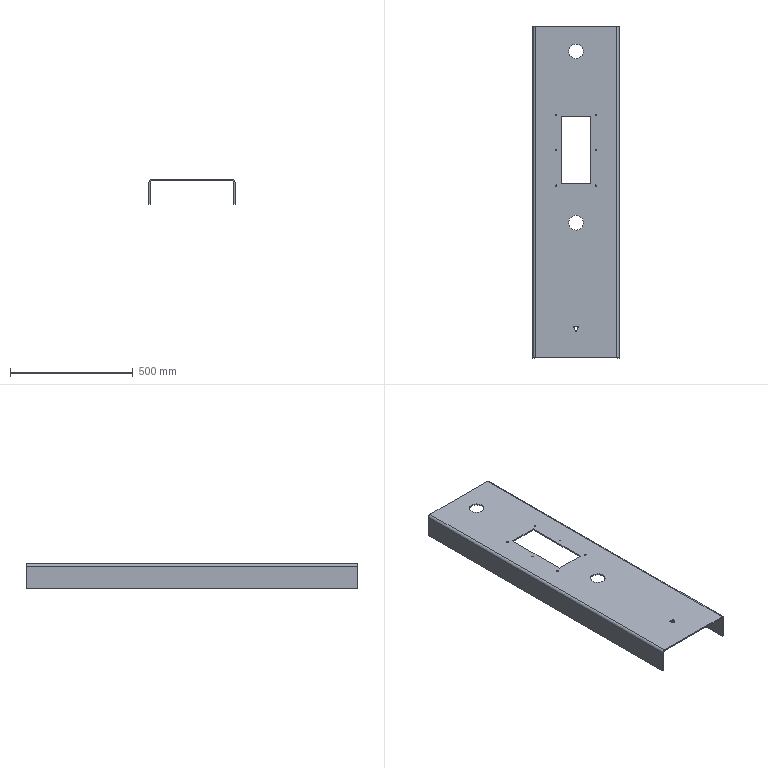Component | SolidWorks | 003FrameFrontWeldingPlate-1 | 1 solid | 46 faces | box 350 x 1350 x 100 mm | volume 3409404 mm3 | cylinder 32 | plane 14 | commonest cylinder face diameters 5 x16 2.5 x6 60 x4 16 x2 20 x2 10 x2 | material Plain Carbon Steel
build123d program:
from build123d import *

# Parameters (mm, degrees)
SKETCH1_W            = 350
SKETCH1_H            = 100
BOSS_EXTRUDE1_DEPTH  = 1350
FILLET1_R            = 10
SHELL1_T             = -5
CUT_EXTRUDE1_REACH   = 1366.963
SKETCH2_W            = 120
SKETCH2_H            = 270
CUT_EXTRUDE2_REACH   = 1366.963
SKETCH3_R            = 30
CUT_EXTRUDE3_REACH   = 1366.963
SKETCH4_R            = 8
LPATTERN1_COUNT      = 2
LPATTERN1_PITCH      = 160
LPATTERN1_COUNT_DIR2 = 3
LPATTERN1_PITCH_DIR2 = 144
LPATTERN2_COUNT      = 2
LPATTERN2_PITCH      = 345
CIRPATTERN1_COUNT    = 3


with BuildPart() as part:
    # Sketch1 → Boss-Extrude1 (new body)
    with BuildSketch(Plane.XY):
        Rectangle(SKETCH1_W, SKETCH1_H)
    extrude(amount=BOSS_EXTRUDE1_DEPTH)

    # Fillet1
    fillet1_edges = [part.edges().sort_by_distance(p)[0] for p in [
        (175, -50, 675),
        (-175, -50, 675),
    ]]
    fillet(fillet1_edges, radius=FILLET1_R)

    # Shell1
    shell1_openings = [part.faces().sort_by_distance(p)[0] for p in [
        (0, 0.05865, 1350),
        (0, 0.05865, 0),
        (0, 50, 675),
    ]]
    offset(amount=SHELL1_T, openings=shell1_openings, kind=Kind.INTERSECTION)

    # Sketch2 → Cut-Extrude1 (cut, up to next)
    with BuildSketch(Plane.XZ.offset(50), mode=Mode.PRIVATE) as cut_extrude1_sk1:
        with Locations((0, 845)):
            Rectangle(SKETCH2_W, SKETCH2_H)
    cut_extrude1_tool1 = extrude(cut_extrude1_sk1.sketch, amount=-CUT_EXTRUDE1_REACH, mode=Mode.PRIVATE) & part.part
    add(cut_extrude1_tool1.solids().sort_by_distance((0, -50, 845))[0], mode=Mode.SUBTRACT)

    # Sketch3 → Cut-Extrude2 (cut, up to next)
    with BuildSketch(Plane.XZ.offset(50), mode=Mode.PRIVATE) as cut_extrude2_sk1:
        with Locations(Location((0, 550, 0), (0, 0, 270))):
            Circle(SKETCH3_R)
    cut_extrude2_tool1 = extrude(cut_extrude2_sk1.sketch, amount=-CUT_EXTRUDE2_REACH, mode=Mode.PRIVATE) & part.part
    # Sketch3 → Cut-Extrude2 (cut, up to next)
    with BuildSketch(Plane.XZ.offset(50), mode=Mode.PRIVATE) as cut_extrude2_sk2:
        with Locations(Location((0, 1246.5, 0), (0, 0, 270))):
            Circle(SKETCH3_R)
    cut_extrude2_tool2 = extrude(cut_extrude2_sk2.sketch, amount=-CUT_EXTRUDE2_REACH, mode=Mode.PRIVATE) & part.part
    add(cut_extrude2_tool1.solids().sort_by_distance((0, -50, 550))[0], mode=Mode.SUBTRACT)
    add(cut_extrude2_tool2.solids().sort_by_distance((0, -50, 1246.5))[0], mode=Mode.SUBTRACT)

    # Sketch4 → Cut-Extrude3 (cut, up to next)
    with BuildSketch(Plane.XZ.offset(50), mode=Mode.PRIVATE) as cut_extrude3_sk1:
        with Locations(Location((0, 120, 0), (0, 0, 270))):
            Circle(SKETCH4_R)
    cut_extrude3_tool1 = extrude(cut_extrude3_sk1.sketch, amount=-CUT_EXTRUDE3_REACH, mode=Mode.PRIVATE) & part.part
    add(cut_extrude3_tool1.solids().sort_by_distance((0, -50, 120))[0], mode=Mode.SUBTRACT)

    # Sketch5 → M6 Tapped Hole1 (revolve, cut)
    with BuildSketch(Plane(origin=(175, 35, 1250), x_dir=(0, 0, -1), z_dir=(0, 1, 0))):
        Polygon((0, 0), (0, 16.502), (2.5, 15), (2.5, 0), align=None)
    m6_tapped_hole1 = revolve(axis=Axis((181.35, 35, 1250), (-1, 0, 0)), mode=Mode.SUBTRACT)

    # Sketch8 → M6 Tapped Hole2 (revolve, cut)
    with BuildSketch(Plane(origin=(-80, -50, 701), x_dir=(0, 0, -1), z_dir=(1, 0, 0))):
        Polygon((0, 0), (0, 16.502), (2.5, 15), (2.5, 0), align=None)
    m6_tapped_hole2 = revolve(axis=Axis((-80, -56.35, 701), (0, 1, 0)), mode=Mode.SUBTRACT)

    # LPattern1: M6 Tapped Hole2 2 × 3
    with Locations(*[(i * LPATTERN1_PITCH, 0, j * LPATTERN1_PITCH_DIR2) for i in range(LPATTERN1_COUNT) for j in range(LPATTERN1_COUNT_DIR2) if (i, j) != (0, 0)]):
        add(m6_tapped_hole2, mode=Mode.SUBTRACT)

    # LPattern2: M6 Tapped Hole1 ×2
    with Locations(*[(0, 0, -i * LPATTERN2_PITCH) for i in range(1, LPATTERN2_COUNT)]):
        add(m6_tapped_hole1, mode=Mode.SUBTRACT)

    # Sketch10 → M3 Tapped Hole1 (revolve, cut)
    with BuildSketch(Plane(origin=(0, -50, 108), x_dir=(0, 0, -1), z_dir=(1, 0, 0))):
        Polygon((0, 0), (0, 8.251), (1.25, 7.5), (1.25, 0), align=None)
    m3_tapped_hole1 = revolve(axis=Axis((0, -56.35, 108), (0, 1, 0)), mode=Mode.SUBTRACT)

    # CirPattern1: M3 Tapped Hole1 ×3 about axis
    cirpattern1_axis = Axis((0, 0, 120), (0, 1, 0))
    for i in range(1, CIRPATTERN1_COUNT):
        add(m3_tapped_hole1.rotate(cirpattern1_axis, i * 360 / CIRPATTERN1_COUNT), mode=Mode.SUBTRACT)


solid = part.part

# Placed as in the assembly
solid = solid.moved(Location((130, 37, -50), (-90, 0, 0)))